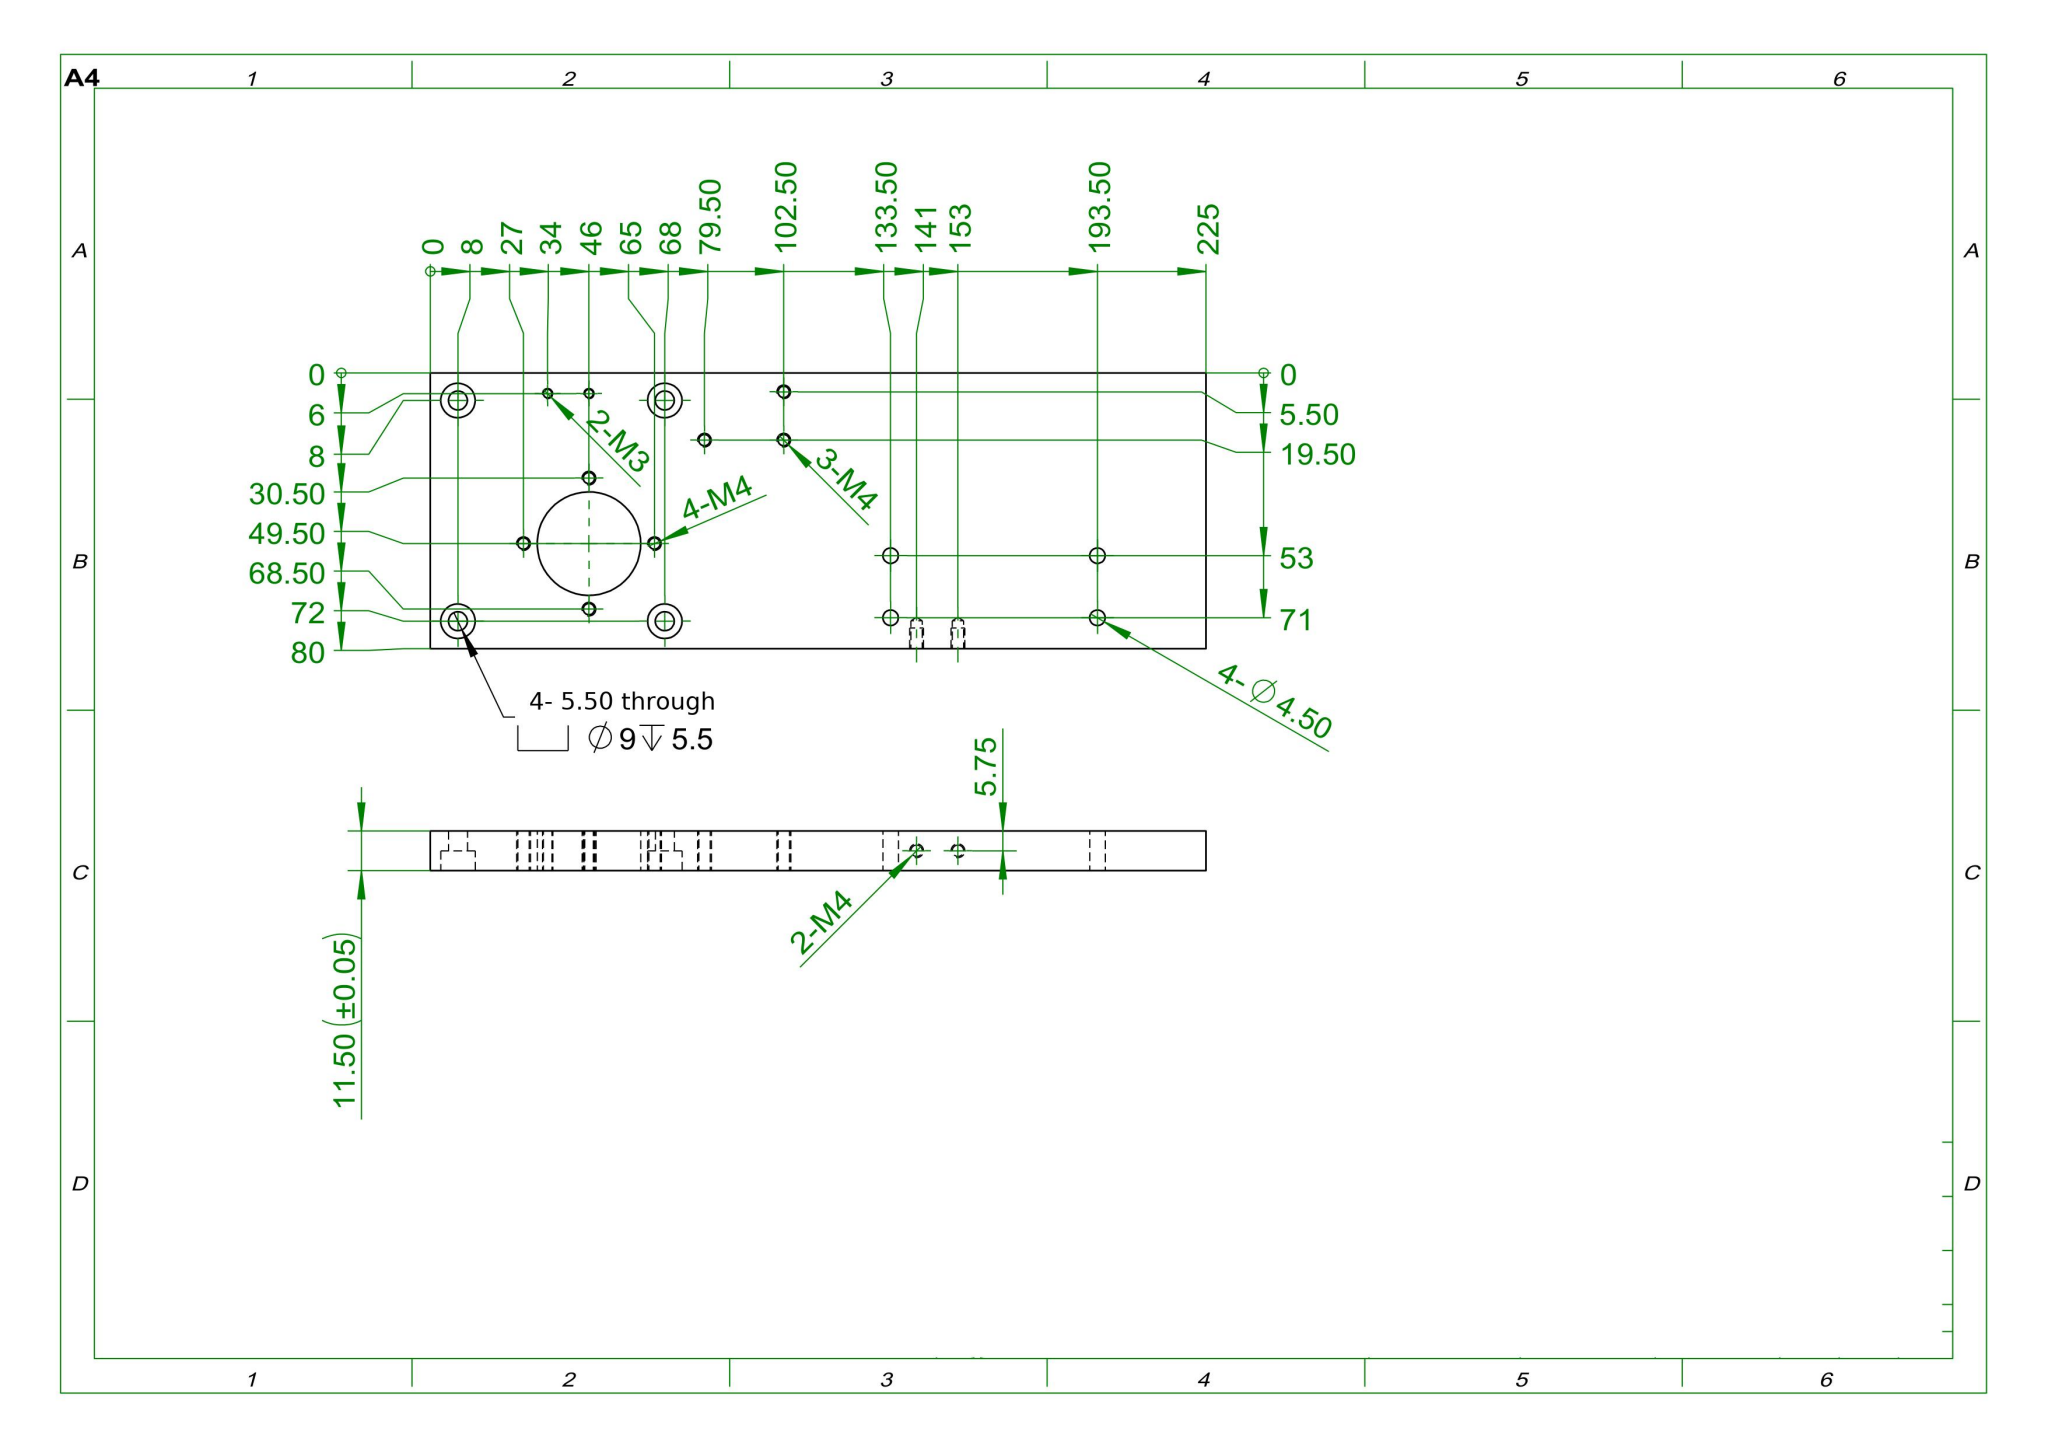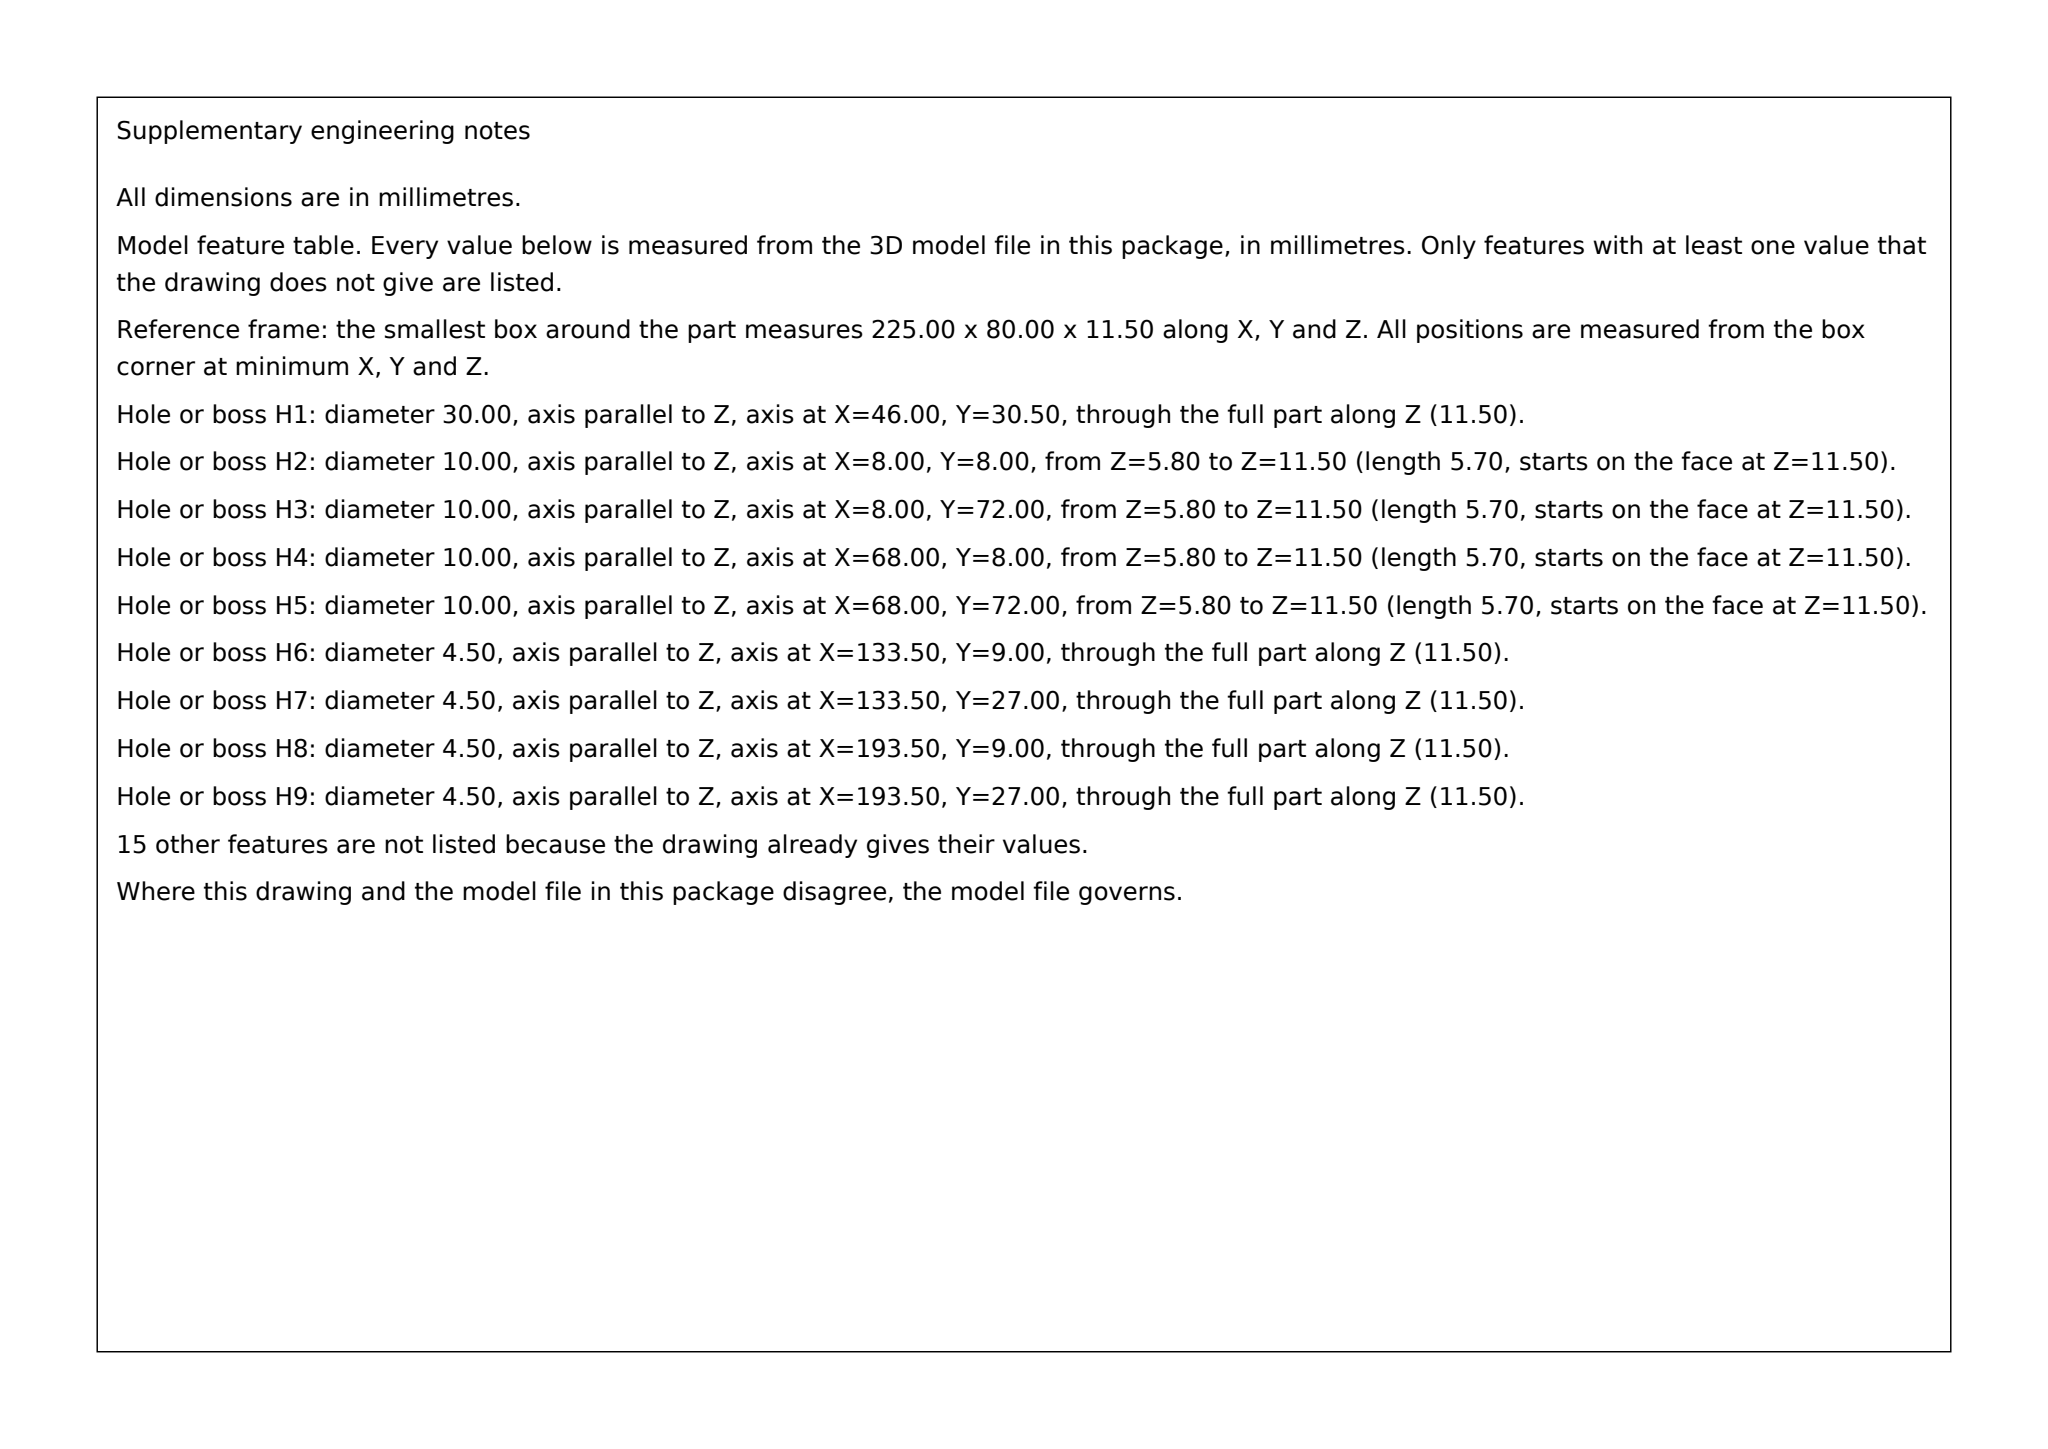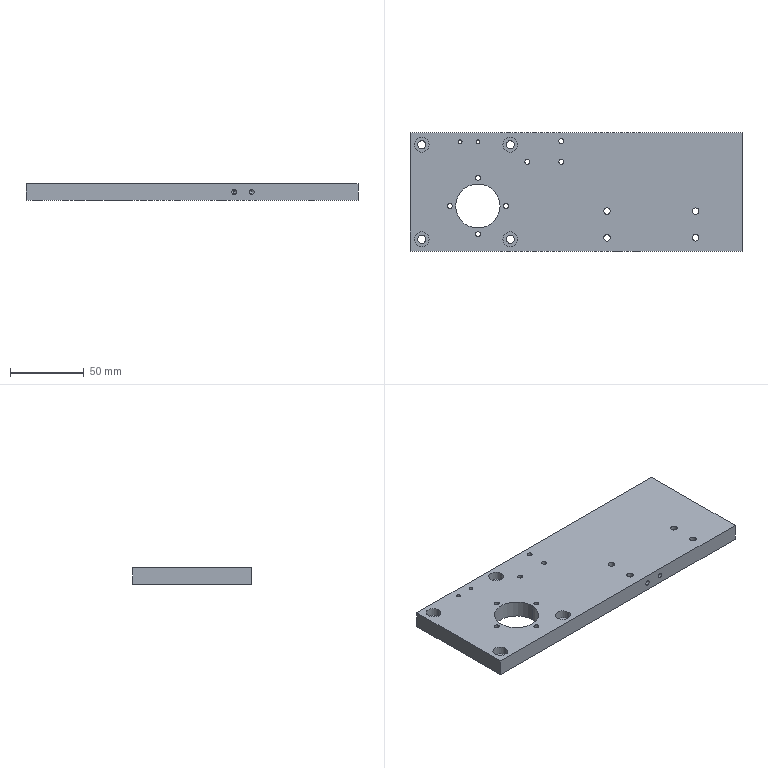Part | SolidWorks | mm | 1 solid | 62 faces | box 225 x 80 x 11.5 mm | volume 194852 mm3 | cylinder 48 | plane 10 | cone 4 | commonest cylinder face diameters 3.3 x18 4.5 x8 10 x8 5.5 x8 2.5 x4 30 x2
build123d program:
from build123d import *

# Parameters (mm, degrees)
SKETCH1_W                                         = 225
SKETCH1_H                                         = 80
BOSS_EXTRUDE1_DEPTH                               = 11.5
HOLE_SIZE_ACCORDING_TO_TYPE_OF_HEXAGO_D           = 5.5
HOLE_SIZE_ACCORDING_TO_TYPE_OF_HEXAGO_CBORE_D     = 10
HOLE_SIZE_ACCORDING_TO_TYPE_OF_HEXAGO_CBORE_DEPTH = 5.7
SKETCH5_R                                         = 15
CUT_EXTRUDE2_DEPTH                                = 20
M4_TAPPED_HOLE1_D                                 = 3.3
F_4_5_4_5_DIAMETER_HOLE1_D                        = 4.5
M4_TAPPED_HOLE2_D                                 = 3.3
M3_TAPPED_HOLE1_D                                 = 2.5
M4_TAPPED_HOLE3_D                                 = 3.3
M4_TAPPED_HOLE3_DEPTH                             = 8.1
M4_TAPPED_HOLE3_TIP                               = 0.9914


with BuildPart() as part:
    # Sketch1 → Boss-Extrude1 (new body)
    with BuildSketch(Plane.XY):
        Rectangle(SKETCH1_W, SKETCH1_H)
    extrude(amount=BOSS_EXTRUDE1_DEPTH)

    # Hole Size _ according to_ Type of Hexago (through all)
    with Locations(Plane.XY.offset(11.5)):
        with Locations((-104.5, 32), (-44.5, 32), (-44.5, -32), (-104.5, -32)):
            CounterBoreHole(HOLE_SIZE_ACCORDING_TO_TYPE_OF_HEXAGO_D / 2, HOLE_SIZE_ACCORDING_TO_TYPE_OF_HEXAGO_CBORE_D / 2, HOLE_SIZE_ACCORDING_TO_TYPE_OF_HEXAGO_CBORE_DEPTH)

    # Sketch5 → Cut-Extrude2 (cut)
    with BuildSketch(Plane.XY.offset(11.5)):
        with Locations((-66.5, -9.5)):
            Circle(SKETCH5_R)
    extrude(amount=-CUT_EXTRUDE2_DEPTH, mode=Mode.SUBTRACT)

    # M4 Tapped Hole1 (through all)
    with Locations(Plane.XY.offset(11.5)):
        with Locations((-10, 20.5), (-10, 34.5), (-33, 20.5)):
            Hole(M4_TAPPED_HOLE1_D / 2)

    # 4.5 _4.5_ Diameter Hole1 (through all)
    with Locations(Plane.XY.offset(11.5)):
        with Locations((21, -13), (81, -13), (81, -31), (21, -31)):
            Hole(F_4_5_4_5_DIAMETER_HOLE1_D / 2)

    # M4 Tapped Hole2 (through all)
    with Locations(Plane.XY.offset(11.5)):
        with Locations((-47.5, -9.5), (-66.5, -28.5), (-85.5, -9.5), (-66.5, 9.5)):
            Hole(M4_TAPPED_HOLE2_D / 2)

    # M3 Tapped Hole1 (through all)
    with Locations(Plane.XY.offset(11.5)):
        with Locations((-66.5, 34), (-78.5, 34)):
            Hole(M3_TAPPED_HOLE1_D / 2)

    # M4 Tapped Hole3
    with Locations(Plane(origin=(0, -40, 0), x_dir=(-1, 0, 0), z_dir=(0, -1, 0))):
        with Locations((-28.5, -5.75), (-40.5, -5.75)):
            Hole(M4_TAPPED_HOLE3_D / 2, depth=M4_TAPPED_HOLE3_DEPTH)
            with Locations((0, 0, -(M4_TAPPED_HOLE3_DEPTH + M4_TAPPED_HOLE3_TIP / 2))):  # 118° drill point
                Cone(0, M4_TAPPED_HOLE3_D / 2, M4_TAPPED_HOLE3_TIP, mode=Mode.SUBTRACT)


solid = part.part